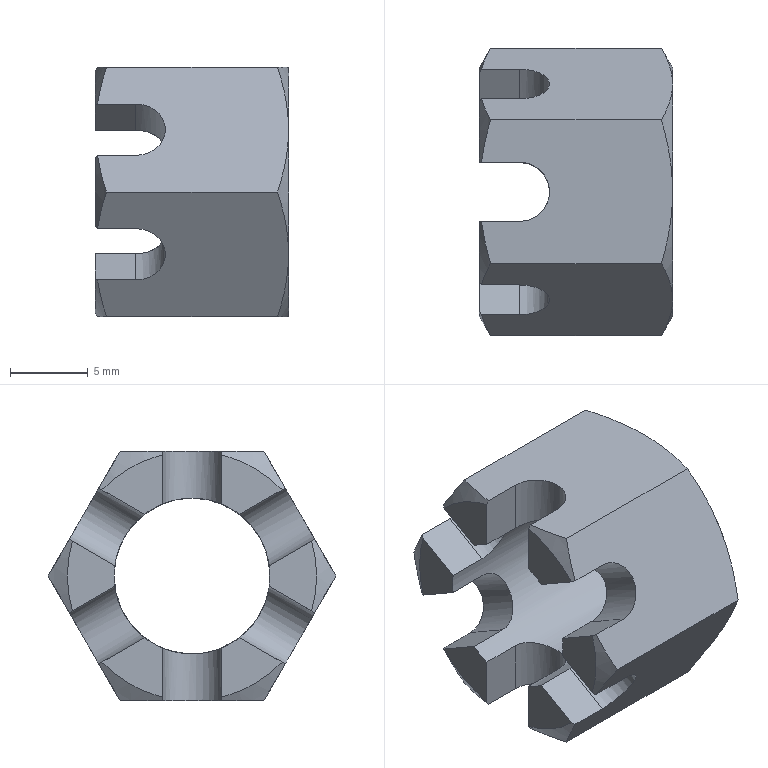Component | NX | 8 | 1 solid | 45 faces | volume 1468 mm3 | plane 25 | cone 13 | cylinder 7 | commonest cylinder face diameters 3.8 x6 10 x1